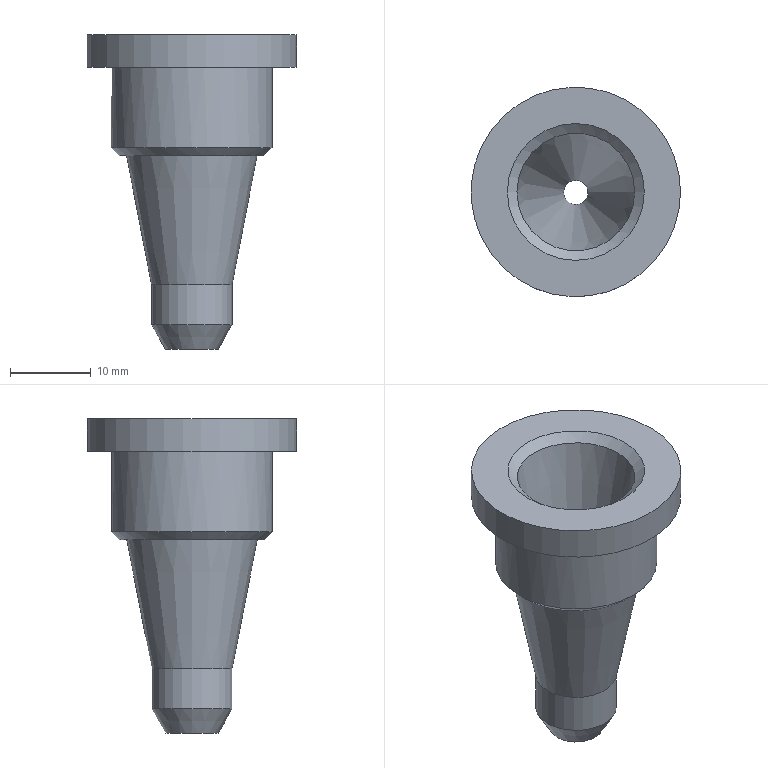Component | NX | SMALL_NOZZLE | 1 solid | 13 faces | box 26 x 26 x 39 mm | volume 5956 mm3 | cone 5 | plane 4 | cylinder 4 | commonest cylinder face diameters 10 x1 3 x1 26 x1 20 x1
STEP:
#1=CARTESIAN_POINT('',(0.,0.,0.));
#2=DIRECTION('',(0.,0.,1.));
#3=DIRECTION('',(1.,0.,0.));
#4=AXIS2_PLACEMENT_3D('',#1,#2,#3);
#5=CARTESIAN_POINT('',(1.284,5.784,7.));
#6=VERTEX_POINT('',#5);
#7=CARTESIAN_POINT('',(10.284,5.784,7.));
#8=DIRECTION('',(0.,0.,-1.));
#9=DIRECTION('',(-1.,0.,0.));
#10=AXIS2_PLACEMENT_3D('',#7,#8,#9);
#11=CIRCLE('',#10,9.);
#12=CARTESIAN_POINT('',(10.284,15.784,7.));
#13=DIRECTION('',(0.,0.,-1.));
#14=DIRECTION('',(-1.,0.,0.));
#15=AXIS2_PLACEMENT_3D('',#12,#13,#14);
#16=PLANE('',#15);
#17=CARTESIAN_POINT('',(0.,-10.));
#18=DIRECTION('',(1.,0.));
#19=AXIS2_PLACEMENT_2D('',#17,#18);
#20=CIRCLE('',#19,9.);
#21=(GEOMETRIC_REPRESENTATION_CONTEXT(2)PARAMETRIC_REPRESENTATION_CONTEXT()REPRESENTATION_CONTEXT('',''));
#22=DEFINITIONAL_REPRESENTATION('',(#20),#21);
#23=PCURVE('',#16,#22);
#24=CARTESIAN_POINT('',(10.284,5.784,8.));
#25=DIRECTION('',(0.,0.,1.));
#26=DIRECTION('',(1.,0.,0.));
#27=AXIS2_PLACEMENT_3D('',#24,#25,#26);
#28=CONICAL_SURFACE('',#27,10.,0.7854);
#29=CARTESIAN_POINT('',(9.425,-1.));
#30=DIRECTION('',(-1.,0.));
#31=VECTOR('',#30,1.);
#32=LINE('',#29,#31);
#33=(GEOMETRIC_REPRESENTATION_CONTEXT(2)PARAMETRIC_REPRESENTATION_CONTEXT()REPRESENTATION_CONTEXT('',''));
#34=DEFINITIONAL_REPRESENTATION('',(#32),#33);
#35=PCURVE('',#28,#34);
#36=SURFACE_CURVE('',#11,(#23,#35),.PCURVE_S1.);
#37=EDGE_CURVE('',#6,#6,#36,.T.);
#38=ORIENTED_EDGE('',*,*,#37,.T.);
#39=EDGE_LOOP('',(#38));
#40=FACE_BOUND('',#39,.T.);
#41=CARTESIAN_POINT('',(18.381,5.784,7.));
#42=VERTEX_POINT('',#41);
#43=CARTESIAN_POINT('',(10.284,5.784,7.));
#44=DIRECTION('',(0.,0.,1.));
#45=DIRECTION('',(1.,0.,0.));
#46=AXIS2_PLACEMENT_3D('',#43,#44,#45);
#47=CIRCLE('',#46,8.097);
#48=CARTESIAN_POINT('',(-8.097,-10.));
#49=CARTESIAN_POINT('',(-8.097,4.024));
#50=CARTESIAN_POINT('',(4.048,-2.988));
#51=CARTESIAN_POINT('',(16.194,-10.));
#52=CARTESIAN_POINT('',(4.048,-17.012));
#53=CARTESIAN_POINT('',(-8.097,-24.024));
#54=CARTESIAN_POINT('',(-8.097,-10.));
#55=(BOUNDED_CURVE()B_SPLINE_CURVE(2,(#48,#49,#50,#51,#52,#53,#54),.UNSPECIFIED.,.T.,.F.)B_SPLINE_CURVE_WITH_KNOTS((1,2,2,2,2,1),(-2.094,0.,2.094,4.189,6.283,8.378),.UNSPECIFIED.)CURVE()GEOMETRIC_REPRESENTATION_ITEM()RATIONAL_B_SPLINE_CURVE((1.,0.5,1.,0.5,1.,0.5,1.))REPRESENTATION_ITEM(''));
#56=(GEOMETRIC_REPRESENTATION_CONTEXT(2)PARAMETRIC_REPRESENTATION_CONTEXT()REPRESENTATION_CONTEXT('',''));
#57=DEFINITIONAL_REPRESENTATION('',(#55),#56);
#58=PCURVE('',#16,#57);
#59=CARTESIAN_POINT('',(10.284,5.784,7.));
#60=DIRECTION('',(0.,0.,1.));
#61=DIRECTION('',(1.,0.,0.));
#62=AXIS2_PLACEMENT_3D('',#59,#60,#61);
#63=CONICAL_SURFACE('',#62,8.097,0.1912);
#64=CARTESIAN_POINT('',(0.,0.));
#65=DIRECTION('',(1.,0.));
#66=VECTOR('',#65,1.);
#67=LINE('',#64,#66);
#68=(GEOMETRIC_REPRESENTATION_CONTEXT(2)PARAMETRIC_REPRESENTATION_CONTEXT()REPRESENTATION_CONTEXT('',''));
#69=DEFINITIONAL_REPRESENTATION('',(#67),#68);
#70=PCURVE('',#63,#69);
#71=SURFACE_CURVE('',#47,(#58,#70),.PCURVE_S1.);
#72=EDGE_CURVE('',#42,#42,#71,.T.);
#73=ORIENTED_EDGE('',*,*,#72,.T.);
#74=EDGE_LOOP('',(#73));
#75=FACE_BOUND('',#74,.T.);
#76=ADVANCED_FACE('',(#40,#75),#16,.T.);
#77=CARTESIAN_POINT('',(15.284,5.784,-9.));
#78=VERTEX_POINT('',#77);
#79=CARTESIAN_POINT('',(10.284,5.784,-9.));
#80=DIRECTION('',(0.,0.,1.));
#81=DIRECTION('',(1.,0.,0.));
#82=AXIS2_PLACEMENT_3D('',#79,#80,#81);
#83=CIRCLE('',#82,5.);
#84=CARTESIAN_POINT('',(0.,-16.));
#85=DIRECTION('',(1.,0.));
#86=VECTOR('',#85,1.);
#87=LINE('',#84,#86);
#88=(GEOMETRIC_REPRESENTATION_CONTEXT(2)PARAMETRIC_REPRESENTATION_CONTEXT()REPRESENTATION_CONTEXT('',''));
#89=DEFINITIONAL_REPRESENTATION('',(#87),#88);
#90=PCURVE('',#63,#89);
#91=CARTESIAN_POINT('',(10.284,5.784,22.));
#92=DIRECTION('',(0.,0.,1.));
#93=DIRECTION('',(1.,0.,0.));
#94=AXIS2_PLACEMENT_3D('',#91,#92,#93);
#95=CYLINDRICAL_SURFACE('',#94,5.);
#96=CARTESIAN_POINT('',(0.,-31.));
#97=DIRECTION('',(1.,0.));
#98=VECTOR('',#97,1.);
#99=LINE('',#96,#98);
#100=(GEOMETRIC_REPRESENTATION_CONTEXT(2)PARAMETRIC_REPRESENTATION_CONTEXT()REPRESENTATION_CONTEXT('',''));
#101=DEFINITIONAL_REPRESENTATION('',(#99),#100);
#102=PCURVE('',#95,#101);
#103=SURFACE_CURVE('',#83,(#90,#102),.PCURVE_S1.);
#104=EDGE_CURVE('',#78,#78,#103,.T.);
#105=ORIENTED_EDGE('',*,*,#104,.T.);
#106=CARTESIAN_POINT('',(15.284,5.784,-9.));
#107=CARTESIAN_POINT('',(18.381,5.784,7.));
#108=B_SPLINE_CURVE_WITH_KNOTS('',1,(#106,#107),.UNSPECIFIED.,.F.,.F.,(2,2),(-16.297,0.),.PIECEWISE_BEZIER_KNOTS.);
#109=CARTESIAN_POINT('',(6.283,0.));
#110=DIRECTION('',(0.,1.));
#111=VECTOR('',#110,1.);
#112=LINE('',#109,#111);
#113=(GEOMETRIC_REPRESENTATION_CONTEXT(2)PARAMETRIC_REPRESENTATION_CONTEXT()REPRESENTATION_CONTEXT('',''));
#114=DEFINITIONAL_REPRESENTATION('',(#112),#113);
#115=PCURVE('',#63,#114);
#116=CARTESIAN_POINT('',(0.,0.));
#117=DIRECTION('',(0.,1.));
#118=VECTOR('',#117,1.);
#119=LINE('',#116,#118);
#120=(GEOMETRIC_REPRESENTATION_CONTEXT(2)PARAMETRIC_REPRESENTATION_CONTEXT()REPRESENTATION_CONTEXT('',''));
#121=DEFINITIONAL_REPRESENTATION('',(#119),#120);
#122=PCURVE('',#63,#121);
#123=SEAM_CURVE('',#108,(#115,#122),.PCURVE_S1.);
#124=EDGE_CURVE('',#78,#42,#123,.T.);
#125=ORIENTED_EDGE('',*,*,#124,.T.);
#126=ORIENTED_EDGE('',*,*,#72,.F.);
#127=ORIENTED_EDGE('',*,*,#124,.F.);
#128=EDGE_LOOP('',(#105,#125,#126,#127));
#129=FACE_BOUND('',#128,.T.);
#130=ADVANCED_FACE('',(#129),#63,.T.);
#131=CARTESIAN_POINT('',(15.284,5.784,-14.));
#132=VERTEX_POINT('',#131);
#133=CARTESIAN_POINT('',(10.284,5.784,-14.));
#134=DIRECTION('',(0.,0.,1.));
#135=DIRECTION('',(1.,0.,0.));
#136=AXIS2_PLACEMENT_3D('',#133,#134,#135);
#137=CIRCLE('',#136,5.);
#138=CARTESIAN_POINT('',(0.,-36.));
#139=DIRECTION('',(1.,0.));
#140=VECTOR('',#139,1.);
#141=LINE('',#138,#140);
#142=(GEOMETRIC_REPRESENTATION_CONTEXT(2)PARAMETRIC_REPRESENTATION_CONTEXT()REPRESENTATION_CONTEXT('',''));
#143=DEFINITIONAL_REPRESENTATION('',(#141),#142);
#144=PCURVE('',#95,#143);
#145=CARTESIAN_POINT('',(10.284,5.784,-14.));
#146=DIRECTION('',(0.,0.,1.));
#147=DIRECTION('',(1.,0.,0.));
#148=AXIS2_PLACEMENT_3D('',#145,#146,#147);
#149=CONICAL_SURFACE('',#148,5.,0.5236);
#150=CARTESIAN_POINT('',(0.,-0.));
#151=DIRECTION('',(1.,0.));
#152=VECTOR('',#151,1.);
#153=LINE('',#150,#152);
#154=(GEOMETRIC_REPRESENTATION_CONTEXT(2)PARAMETRIC_REPRESENTATION_CONTEXT()REPRESENTATION_CONTEXT('',''));
#155=DEFINITIONAL_REPRESENTATION('',(#153),#154);
#156=PCURVE('',#149,#155);
#157=SURFACE_CURVE('',#137,(#144,#156),.PCURVE_S1.);
#158=EDGE_CURVE('',#132,#132,#157,.T.);
#159=ORIENTED_EDGE('',*,*,#158,.T.);
#160=CARTESIAN_POINT('',(15.284,5.784,-14.));
#161=CARTESIAN_POINT('',(15.284,5.784,-9.));
#162=B_SPLINE_CURVE_WITH_KNOTS('',1,(#160,#161),.UNSPECIFIED.,.F.,.F.,(2,2),(-36.,-31.),.PIECEWISE_BEZIER_KNOTS.);
#163=CARTESIAN_POINT('',(6.283,0.));
#164=DIRECTION('',(0.,1.));
#165=VECTOR('',#164,1.);
#166=LINE('',#163,#165);
#167=(GEOMETRIC_REPRESENTATION_CONTEXT(2)PARAMETRIC_REPRESENTATION_CONTEXT()REPRESENTATION_CONTEXT('',''));
#168=DEFINITIONAL_REPRESENTATION('',(#166),#167);
#169=PCURVE('',#95,#168);
#170=CARTESIAN_POINT('',(0.,0.));
#171=DIRECTION('',(0.,1.));
#172=VECTOR('',#171,1.);
#173=LINE('',#170,#172);
#174=(GEOMETRIC_REPRESENTATION_CONTEXT(2)PARAMETRIC_REPRESENTATION_CONTEXT()REPRESENTATION_CONTEXT('',''));
#175=DEFINITIONAL_REPRESENTATION('',(#173),#174);
#176=PCURVE('',#95,#175);
#177=SEAM_CURVE('',#162,(#169,#176),.PCURVE_S1.);
#178=EDGE_CURVE('',#132,#78,#177,.T.);
#179=ORIENTED_EDGE('',*,*,#178,.T.);
#180=ORIENTED_EDGE('',*,*,#104,.F.);
#181=ORIENTED_EDGE('',*,*,#178,.F.);
#182=EDGE_LOOP('',(#159,#179,#180,#181));
#183=FACE_BOUND('',#182,.T.);
#184=ADVANCED_FACE('',(#183),#95,.T.);
#185=CARTESIAN_POINT('',(13.552,5.784,-17.));
#186=VERTEX_POINT('',#185);
#187=CARTESIAN_POINT('',(10.284,5.784,-17.));
#188=DIRECTION('',(0.,0.,1.));
#189=DIRECTION('',(1.,0.,0.));
#190=AXIS2_PLACEMENT_3D('',#187,#188,#189);
#191=CIRCLE('',#190,3.268);
#192=CARTESIAN_POINT('',(0.,-3.));
#193=DIRECTION('',(1.,0.));
#194=VECTOR('',#193,1.);
#195=LINE('',#192,#194);
#196=(GEOMETRIC_REPRESENTATION_CONTEXT(2)PARAMETRIC_REPRESENTATION_CONTEXT()REPRESENTATION_CONTEXT('',''));
#197=DEFINITIONAL_REPRESENTATION('',(#195),#196);
#198=PCURVE('',#149,#197);
#199=CARTESIAN_POINT('',(10.284,9.052,-17.));
#200=DIRECTION('',(0.,0.,-1.));
#201=DIRECTION('',(-1.,0.,0.));
#202=AXIS2_PLACEMENT_3D('',#199,#200,#201);
#203=PLANE('',#202);
#204=CARTESIAN_POINT('',(-3.268,-3.268));
#205=CARTESIAN_POINT('',(-3.268,2.392));
#206=CARTESIAN_POINT('',(1.634,-0.4378));
#207=CARTESIAN_POINT('',(6.536,-3.268));
#208=CARTESIAN_POINT('',(1.634,-6.098));
#209=CARTESIAN_POINT('',(-3.268,-8.928));
#210=CARTESIAN_POINT('',(-3.268,-3.268));
#211=(BOUNDED_CURVE()B_SPLINE_CURVE(2,(#204,#205,#206,#207,#208,#209,#210),.UNSPECIFIED.,.T.,.F.)B_SPLINE_CURVE_WITH_KNOTS((1,2,2,2,2,1),(-2.094,0.,2.094,4.189,6.283,8.378),.UNSPECIFIED.)CURVE()GEOMETRIC_REPRESENTATION_ITEM()RATIONAL_B_SPLINE_CURVE((1.,0.5,1.,0.5,1.,0.5,1.))REPRESENTATION_ITEM(''));
#212=(GEOMETRIC_REPRESENTATION_CONTEXT(2)PARAMETRIC_REPRESENTATION_CONTEXT()REPRESENTATION_CONTEXT('',''));
#213=DEFINITIONAL_REPRESENTATION('',(#211),#212);
#214=PCURVE('',#203,#213);
#215=SURFACE_CURVE('',#191,(#198,#214),.PCURVE_S1.);
#216=EDGE_CURVE('',#186,#186,#215,.T.);
#217=ORIENTED_EDGE('',*,*,#216,.T.);
#218=CARTESIAN_POINT('',(13.552,5.784,-17.));
#219=CARTESIAN_POINT('',(15.284,5.784,-14.));
#220=B_SPLINE_CURVE_WITH_KNOTS('',1,(#218,#219),.UNSPECIFIED.,.F.,.F.,(2,2),(-3.464,-0.),.PIECEWISE_BEZIER_KNOTS.);
#221=CARTESIAN_POINT('',(6.283,0.));
#222=DIRECTION('',(0.,1.));
#223=VECTOR('',#222,1.);
#224=LINE('',#221,#223);
#225=(GEOMETRIC_REPRESENTATION_CONTEXT(2)PARAMETRIC_REPRESENTATION_CONTEXT()REPRESENTATION_CONTEXT('',''));
#226=DEFINITIONAL_REPRESENTATION('',(#224),#225);
#227=PCURVE('',#149,#226);
#228=CARTESIAN_POINT('',(0.,0.));
#229=DIRECTION('',(0.,1.));
#230=VECTOR('',#229,1.);
#231=LINE('',#228,#230);
#232=(GEOMETRIC_REPRESENTATION_CONTEXT(2)PARAMETRIC_REPRESENTATION_CONTEXT()REPRESENTATION_CONTEXT('',''));
#233=DEFINITIONAL_REPRESENTATION('',(#231),#232);
#234=PCURVE('',#149,#233);
#235=SEAM_CURVE('',#220,(#227,#234),.PCURVE_S1.);
#236=EDGE_CURVE('',#186,#132,#235,.T.);
#237=ORIENTED_EDGE('',*,*,#236,.T.);
#238=ORIENTED_EDGE('',*,*,#158,.F.);
#239=ORIENTED_EDGE('',*,*,#236,.F.);
#240=EDGE_LOOP('',(#217,#237,#238,#239));
#241=FACE_BOUND('',#240,.T.);
#242=ADVANCED_FACE('',(#241),#149,.T.);
#243=CARTESIAN_POINT('',(11.784,5.784,-17.));
#244=VERTEX_POINT('',#243);
#245=CARTESIAN_POINT('',(10.284,5.784,-17.));
#246=DIRECTION('',(0.,0.,1.));
#247=DIRECTION('',(1.,0.,0.));
#248=AXIS2_PLACEMENT_3D('',#245,#246,#247);
#249=CIRCLE('',#248,1.5);
#250=CARTESIAN_POINT('',(-1.5,-3.268));
#251=CARTESIAN_POINT('',(-1.5,-0.6699));
#252=CARTESIAN_POINT('',(0.75,-1.969));
#253=CARTESIAN_POINT('',(3.,-3.268));
#254=CARTESIAN_POINT('',(0.75,-4.567));
#255=CARTESIAN_POINT('',(-1.5,-5.866));
#256=CARTESIAN_POINT('',(-1.5,-3.268));
#257=(BOUNDED_CURVE()B_SPLINE_CURVE(2,(#250,#251,#252,#253,#254,#255,#256),.UNSPECIFIED.,.T.,.F.)B_SPLINE_CURVE_WITH_KNOTS((1,2,2,2,2,1),(-2.094,0.,2.094,4.189,6.283,8.378),.UNSPECIFIED.)CURVE()GEOMETRIC_REPRESENTATION_ITEM()RATIONAL_B_SPLINE_CURVE((1.,0.5,1.,0.5,1.,0.5,1.))REPRESENTATION_ITEM(''));
#258=(GEOMETRIC_REPRESENTATION_CONTEXT(2)PARAMETRIC_REPRESENTATION_CONTEXT()REPRESENTATION_CONTEXT('',''));
#259=DEFINITIONAL_REPRESENTATION('',(#257),#258);
#260=PCURVE('',#203,#259);
#261=CARTESIAN_POINT('',(10.284,5.784,22.));
#262=DIRECTION('',(0.,0.,1.));
#263=DIRECTION('',(1.,0.,0.));
#264=AXIS2_PLACEMENT_3D('',#261,#262,#263);
#265=CYLINDRICAL_SURFACE('',#264,1.5);
#266=CARTESIAN_POINT('',(0.,-39.));
#267=DIRECTION('',(1.,0.));
#268=VECTOR('',#267,1.);
#269=LINE('',#266,#268);
#270=(GEOMETRIC_REPRESENTATION_CONTEXT(2)PARAMETRIC_REPRESENTATION_CONTEXT()REPRESENTATION_CONTEXT('',''));
#271=DEFINITIONAL_REPRESENTATION('',(#269),#270);
#272=PCURVE('',#265,#271);
#273=SURFACE_CURVE('',#249,(#260,#272),.PCURVE_S1.);
#274=EDGE_CURVE('',#244,#244,#273,.T.);
#275=ORIENTED_EDGE('',*,*,#274,.T.);
#276=EDGE_LOOP('',(#275));
#277=FACE_BOUND('',#276,.T.);
#278=ORIENTED_EDGE('',*,*,#216,.F.);
#279=EDGE_LOOP('',(#278));
#280=FACE_BOUND('',#279,.T.);
#281=ADVANCED_FACE('',(#277,#280),#203,.T.);
#282=CARTESIAN_POINT('',(11.784,5.784,-9.));
#283=VERTEX_POINT('',#282);
#284=CARTESIAN_POINT('',(10.284,5.784,-9.));
#285=DIRECTION('',(0.,0.,1.));
#286=DIRECTION('',(1.,0.,0.));
#287=AXIS2_PLACEMENT_3D('',#284,#285,#286);
#288=CIRCLE('',#287,1.5);
#289=CARTESIAN_POINT('',(0.,-31.));
#290=DIRECTION('',(1.,0.));
#291=VECTOR('',#290,1.);
#292=LINE('',#289,#291);
#293=(GEOMETRIC_REPRESENTATION_CONTEXT(2)PARAMETRIC_REPRESENTATION_CONTEXT()REPRESENTATION_CONTEXT('',''));
#294=DEFINITIONAL_REPRESENTATION('',(#292),#293);
#295=PCURVE('',#265,#294);
#296=CARTESIAN_POINT('',(10.284,5.784,-9.));
#297=DIRECTION('',(0.,0.,1.));
#298=DIRECTION('',(1.,0.,0.));
#299=AXIS2_PLACEMENT_3D('',#296,#297,#298);
#300=CONICAL_SURFACE('',#299,1.5,0.1912);
#301=CARTESIAN_POINT('',(0.,0.));
#302=DIRECTION('',(1.,0.));
#303=VECTOR('',#302,1.);
#304=LINE('',#301,#303);
#305=(GEOMETRIC_REPRESENTATION_CONTEXT(2)PARAMETRIC_REPRESENTATION_CONTEXT()REPRESENTATION_CONTEXT('',''));
#306=DEFINITIONAL_REPRESENTATION('',(#304),#305);
#307=PCURVE('',#300,#306);
#308=SURFACE_CURVE('',#288,(#295,#307),.PCURVE_S1.);
#309=EDGE_CURVE('',#283,#283,#308,.T.);
#310=ORIENTED_EDGE('',*,*,#309,.F.);
#311=CARTESIAN_POINT('',(11.784,5.784,-17.));
#312=CARTESIAN_POINT('',(11.784,5.784,-9.));
#313=B_SPLINE_CURVE_WITH_KNOTS('',1,(#311,#312),.UNSPECIFIED.,.F.,.F.,(2,2),(-39.,-31.),.PIECEWISE_BEZIER_KNOTS.);
#314=CARTESIAN_POINT('',(0.,0.));
#315=DIRECTION('',(0.,1.));
#316=VECTOR('',#315,1.);
#317=LINE('',#314,#316);
#318=(GEOMETRIC_REPRESENTATION_CONTEXT(2)PARAMETRIC_REPRESENTATION_CONTEXT()REPRESENTATION_CONTEXT('',''));
#319=DEFINITIONAL_REPRESENTATION('',(#317),#318);
#320=PCURVE('',#265,#319);
#321=CARTESIAN_POINT('',(6.283,0.));
#322=DIRECTION('',(0.,1.));
#323=VECTOR('',#322,1.);
#324=LINE('',#321,#323);
#325=(GEOMETRIC_REPRESENTATION_CONTEXT(2)PARAMETRIC_REPRESENTATION_CONTEXT()REPRESENTATION_CONTEXT('',''));
#326=DEFINITIONAL_REPRESENTATION('',(#324),#325);
#327=PCURVE('',#265,#326);
#328=SEAM_CURVE('',#313,(#320,#327),.PCURVE_S1.);
#329=EDGE_CURVE('',#244,#283,#328,.T.);
#330=ORIENTED_EDGE('',*,*,#329,.F.);
#331=ORIENTED_EDGE('',*,*,#274,.T.);
#332=ORIENTED_EDGE('',*,*,#329,.T.);
#333=EDGE_LOOP('',(#310,#330,#331,#332));
#334=FACE_BOUND('',#333,.F.);
#335=ADVANCED_FACE('',(#334),#265,.F.);
#336=CARTESIAN_POINT('',(17.594,5.784,21.018));
#337=VERTEX_POINT('',#336);
#338=CARTESIAN_POINT('',(2.974,5.784,21.018));
#339=VERTEX_POINT('',#338);
#340=CARTESIAN_POINT('',(10.284,5.784,21.018));
#341=DIRECTION('',(0.,0.,1.));
#342=DIRECTION('',(-1.,0.,0.));
#343=AXIS2_PLACEMENT_3D('',#340,#341,#342);
#344=CIRCLE('',#343,7.31);
#345=CARTESIAN_POINT('',(-3.142,30.018));
#346=DIRECTION('',(1.,0.));
#347=VECTOR('',#346,1.);
#348=LINE('',#345,#347);
#349=(GEOMETRIC_REPRESENTATION_CONTEXT(2)PARAMETRIC_REPRESENTATION_CONTEXT()REPRESENTATION_CONTEXT('',''));
#350=DEFINITIONAL_REPRESENTATION('',(#348),#349);
#351=PCURVE('',#300,#350);
#352=CARTESIAN_POINT('',(10.284,5.784,21.018));
#353=DIRECTION('',(0.,0.,1.));
#354=DIRECTION('',(1.,0.,0.));
#355=AXIS2_PLACEMENT_3D('',#352,#353,#354);
#356=CONICAL_SURFACE('',#355,7.31,0.881);
#357=CARTESIAN_POINT('',(-3.142,0.));
#358=DIRECTION('',(1.,-0.));
#359=VECTOR('',#358,1.);
#360=LINE('',#357,#359);
#361=(GEOMETRIC_REPRESENTATION_CONTEXT(2)PARAMETRIC_REPRESENTATION_CONTEXT()REPRESENTATION_CONTEXT('',''));
#362=DEFINITIONAL_REPRESENTATION('',(#360),#361);
#363=PCURVE('',#356,#362);
#364=SURFACE_CURVE('',#344,(#351,#363),.PCURVE_S1.);
#365=EDGE_CURVE('',#337,#339,#364,.T.);
#366=ORIENTED_EDGE('',*,*,#365,.F.);
#367=CARTESIAN_POINT('',(11.784,5.784,-9.));
#368=CARTESIAN_POINT('',(17.594,5.784,21.018));
#369=B_SPLINE_CURVE_WITH_KNOTS('',1,(#367,#368),.UNSPECIFIED.,.F.,.F.,(2,2),(0.,30.575),.PIECEWISE_BEZIER_KNOTS.);
#370=CARTESIAN_POINT('',(0.,0.));
#371=DIRECTION('',(0.,1.));
#372=VECTOR('',#371,1.);
#373=LINE('',#370,#372);
#374=(GEOMETRIC_REPRESENTATION_CONTEXT(2)PARAMETRIC_REPRESENTATION_CONTEXT()REPRESENTATION_CONTEXT('',''));
#375=DEFINITIONAL_REPRESENTATION('',(#373),#374);
#376=PCURVE('',#300,#375);
#377=CARTESIAN_POINT('',(6.283,0.));
#378=DIRECTION('',(0.,1.));
#379=VECTOR('',#378,1.);
#380=LINE('',#377,#379);
#381=(GEOMETRIC_REPRESENTATION_CONTEXT(2)PARAMETRIC_REPRESENTATION_CONTEXT()REPRESENTATION_CONTEXT('',''));
#382=DEFINITIONAL_REPRESENTATION('',(#380),#381);
#383=PCURVE('',#300,#382);
#384=SEAM_CURVE('',#369,(#376,#383),.PCURVE_S1.);
#385=EDGE_CURVE('',#283,#337,#384,.T.);
#386=ORIENTED_EDGE('',*,*,#385,.F.);
#387=ORIENTED_EDGE('',*,*,#309,.T.);
#388=ORIENTED_EDGE('',*,*,#385,.T.);
#389=CARTESIAN_POINT('',(10.284,5.784,21.018));
#390=DIRECTION('',(0.,0.,1.));
#391=DIRECTION('',(-1.,0.,0.));
#392=AXIS2_PLACEMENT_3D('',#389,#390,#391);
#393=CIRCLE('',#392,7.31);
#394=CARTESIAN_POINT('',(3.142,30.018));
#395=DIRECTION('',(1.,0.));
#396=VECTOR('',#395,1.);
#397=LINE('',#394,#396);
#398=(GEOMETRIC_REPRESENTATION_CONTEXT(2)PARAMETRIC_REPRESENTATION_CONTEXT()REPRESENTATION_CONTEXT('',''));
#399=DEFINITIONAL_REPRESENTATION('',(#397),#398);
#400=PCURVE('',#300,#399);
#401=CARTESIAN_POINT('',(3.142,0.));
#402=DIRECTION('',(1.,0.));
#403=VECTOR('',#402,1.);
#404=LINE('',#401,#403);
#405=(GEOMETRIC_REPRESENTATION_CONTEXT(2)PARAMETRIC_REPRESENTATION_CONTEXT()REPRESENTATION_CONTEXT('',''));
#406=DEFINITIONAL_REPRESENTATION('',(#404),#405);
#407=PCURVE('',#356,#406);
#408=SURFACE_CURVE('',#393,(#400,#407),.PCURVE_S1.);
#409=EDGE_CURVE('',#339,#337,#408,.T.);
#410=ORIENTED_EDGE('',*,*,#409,.F.);
#411=EDGE_LOOP('',(#366,#386,#387,#388,#410));
#412=FACE_BOUND('',#411,.F.);
#413=ADVANCED_FACE('',(#412),#300,.F.);
#414=CARTESIAN_POINT('',(18.784,5.784,22.));
#415=VERTEX_POINT('',#414);
#416=CARTESIAN_POINT('',(10.284,5.784,22.));
#417=DIRECTION('',(0.,0.,-1.));
#418=DIRECTION('',(1.,0.,0.));
#419=AXIS2_PLACEMENT_3D('',#416,#417,#418);
#420=CIRCLE('',#419,8.5);
#421=CARTESIAN_POINT('',(10.284,13.284,22.));
#422=DIRECTION('',(0.,0.,1.));
#423=DIRECTION('',(1.,0.,0.));
#424=AXIS2_PLACEMENT_3D('',#421,#422,#423);
#425=PLANE('',#424);
#426=CARTESIAN_POINT('',(8.5,-7.5));
#427=CARTESIAN_POINT('',(8.5,-22.222));
#428=CARTESIAN_POINT('',(-4.25,-14.861));
#429=CARTESIAN_POINT('',(-17.,-7.5));
#430=CARTESIAN_POINT('',(-4.25,-0.1388));
#431=CARTESIAN_POINT('',(8.5,7.222));
#432=CARTESIAN_POINT('',(8.5,-7.5));
#433=(BOUNDED_CURVE()B_SPLINE_CURVE(2,(#426,#427,#428,#429,#430,#431,#432),.UNSPECIFIED.,.T.,.F.)B_SPLINE_CURVE_WITH_KNOTS((1,2,2,2,2,1),(-2.094,0.,2.094,4.189,6.283,8.378),.UNSPECIFIED.)CURVE()GEOMETRIC_REPRESENTATION_ITEM()RATIONAL_B_SPLINE_CURVE((1.,0.5,1.,0.5,1.,0.5,1.))REPRESENTATION_ITEM(''));
#434=(GEOMETRIC_REPRESENTATION_CONTEXT(2)PARAMETRIC_REPRESENTATION_CONTEXT()REPRESENTATION_CONTEXT('',''));
#435=DEFINITIONAL_REPRESENTATION('',(#433),#434);
#436=PCURVE('',#425,#435);
#437=CARTESIAN_POINT('',(6.283,0.9818));
#438=DIRECTION('',(-1.,0.));
#439=VECTOR('',#438,1.);
#440=LINE('',#437,#439);
#441=(GEOMETRIC_REPRESENTATION_CONTEXT(2)PARAMETRIC_REPRESENTATION_CONTEXT()REPRESENTATION_CONTEXT('',''));
#442=DEFINITIONAL_REPRESENTATION('',(#440),#441);
#443=PCURVE('',#356,#442);
#444=SURFACE_CURVE('',#420,(#436,#443),.PCURVE_S1.);
#445=EDGE_CURVE('',#415,#415,#444,.T.);
#446=ORIENTED_EDGE('',*,*,#445,.T.);
#447=EDGE_LOOP('',(#446));
#448=FACE_BOUND('',#447,.T.);
#449=CARTESIAN_POINT('',(23.284,5.784,22.));
#450=VERTEX_POINT('',#449);
#451=CARTESIAN_POINT('',(10.284,5.784,22.));
#452=DIRECTION('',(0.,0.,1.));
#453=DIRECTION('',(1.,0.,0.));
#454=AXIS2_PLACEMENT_3D('',#451,#452,#453);
#455=CIRCLE('',#454,13.);
#456=CARTESIAN_POINT('',(0.,-7.5));
#457=DIRECTION('',(1.,0.));
#458=AXIS2_PLACEMENT_2D('',#456,#457);
#459=CIRCLE('',#458,13.);
#460=(GEOMETRIC_REPRESENTATION_CONTEXT(2)PARAMETRIC_REPRESENTATION_CONTEXT()REPRESENTATION_CONTEXT('',''));
#461=DEFINITIONAL_REPRESENTATION('',(#459),#460);
#462=PCURVE('',#425,#461);
#463=CARTESIAN_POINT('',(10.284,5.784,22.));
#464=DIRECTION('',(0.,0.,1.));
#465=DIRECTION('',(1.,0.,0.));
#466=AXIS2_PLACEMENT_3D('',#463,#464,#465);
#467=CYLINDRICAL_SURFACE('',#466,13.);
#468=CARTESIAN_POINT('',(0.,0.));
#469=DIRECTION('',(1.,0.));
#470=VECTOR('',#469,1.);
#471=LINE('',#468,#470);
#472=(GEOMETRIC_REPRESENTATION_CONTEXT(2)PARAMETRIC_REPRESENTATION_CONTEXT()REPRESENTATION_CONTEXT('',''));
#473=DEFINITIONAL_REPRESENTATION('',(#471),#472);
#474=PCURVE('',#467,#473);
#475=SURFACE_CURVE('',#455,(#462,#474),.PCURVE_S1.);
#476=EDGE_CURVE('',#450,#450,#475,.T.);
#477=ORIENTED_EDGE('',*,*,#476,.T.);
#478=EDGE_LOOP('',(#477));
#479=FACE_BOUND('',#478,.T.);
#480=ADVANCED_FACE('',(#448,#479),#425,.T.);
#481=CARTESIAN_POINT('',(23.284,5.784,18.));
#482=VERTEX_POINT('',#481);
#483=CARTESIAN_POINT('',(10.284,5.784,18.));
#484=DIRECTION('',(0.,0.,1.));
#485=DIRECTION('',(1.,0.,0.));
#486=AXIS2_PLACEMENT_3D('',#483,#484,#485);
#487=CIRCLE('',#486,13.);
#488=CARTESIAN_POINT('',(0.,-4.));
#489=DIRECTION('',(1.,0.));
#490=VECTOR('',#489,1.);
#491=LINE('',#488,#490);
#492=(GEOMETRIC_REPRESENTATION_CONTEXT(2)PARAMETRIC_REPRESENTATION_CONTEXT()REPRESENTATION_CONTEXT('',''));
#493=DEFINITIONAL_REPRESENTATION('',(#491),#492);
#494=PCURVE('',#467,#493);
#495=CARTESIAN_POINT('',(10.284,18.784,18.));
#496=DIRECTION('',(0.,0.,-1.));
#497=DIRECTION('',(-1.,0.,0.));
#498=AXIS2_PLACEMENT_3D('',#495,#496,#497);
#499=PLANE('',#498);
#500=CARTESIAN_POINT('',(-13.,-13.));
#501=CARTESIAN_POINT('',(-13.,9.517));
#502=CARTESIAN_POINT('',(6.5,-1.742));
#503=CARTESIAN_POINT('',(26.,-13.));
#504=CARTESIAN_POINT('',(6.5,-24.258));
#505=CARTESIAN_POINT('',(-13.,-35.517));
#506=CARTESIAN_POINT('',(-13.,-13.));
#507=(BOUNDED_CURVE()B_SPLINE_CURVE(2,(#500,#501,#502,#503,#504,#505,#506),.UNSPECIFIED.,.T.,.F.)B_SPLINE_CURVE_WITH_KNOTS((1,2,2,2,2,1),(-2.094,0.,2.094,4.189,6.283,8.378),.UNSPECIFIED.)CURVE()GEOMETRIC_REPRESENTATION_ITEM()RATIONAL_B_SPLINE_CURVE((1.,0.5,1.,0.5,1.,0.5,1.))REPRESENTATION_ITEM(''));
#508=(GEOMETRIC_REPRESENTATION_CONTEXT(2)PARAMETRIC_REPRESENTATION_CONTEXT()REPRESENTATION_CONTEXT('',''));
#509=DEFINITIONAL_REPRESENTATION('',(#507),#508);
#510=PCURVE('',#499,#509);
#511=SURFACE_CURVE('',#487,(#494,#510),.PCURVE_S1.);
#512=EDGE_CURVE('',#482,#482,#511,.T.);
#513=ORIENTED_EDGE('',*,*,#512,.T.);
#514=CARTESIAN_POINT('',(23.284,5.784,18.));
#515=CARTESIAN_POINT('',(23.284,5.784,22.));
#516=B_SPLINE_CURVE_WITH_KNOTS('',1,(#514,#515),.UNSPECIFIED.,.F.,.F.,(2,2),(-4.,0.),.PIECEWISE_BEZIER_KNOTS.);
#517=CARTESIAN_POINT('',(6.283,0.));
#518=DIRECTION('',(0.,1.));
#519=VECTOR('',#518,1.);
#520=LINE('',#517,#519);
#521=(GEOMETRIC_REPRESENTATION_CONTEXT(2)PARAMETRIC_REPRESENTATION_CONTEXT()REPRESENTATION_CONTEXT('',''));
#522=DEFINITIONAL_REPRESENTATION('',(#520),#521);
#523=PCURVE('',#467,#522);
#524=CARTESIAN_POINT('',(0.,0.));
#525=DIRECTION('',(0.,1.));
#526=VECTOR('',#525,1.);
#527=LINE('',#524,#526);
#528=(GEOMETRIC_REPRESENTATION_CONTEXT(2)PARAMETRIC_REPRESENTATION_CONTEXT()REPRESENTATION_CONTEXT('',''));
#529=DEFINITIONAL_REPRESENTATION('',(#527),#528);
#530=PCURVE('',#467,#529);
#531=SEAM_CURVE('',#516,(#523,#530),.PCURVE_S1.);
#532=EDGE_CURVE('',#482,#450,#531,.T.);
#533=ORIENTED_EDGE('',*,*,#532,.T.);
#534=ORIENTED_EDGE('',*,*,#476,.F.);
#535=ORIENTED_EDGE('',*,*,#532,.F.);
#536=EDGE_LOOP('',(#513,#533,#534,#535));
#537=FACE_BOUND('',#536,.T.);
#538=ADVANCED_FACE('',(#537),#467,.T.);
#539=CARTESIAN_POINT('',(20.284,5.784,18.));
#540=VERTEX_POINT('',#539);
#541=CARTESIAN_POINT('',(10.284,5.784,18.));
#542=DIRECTION('',(0.,0.,1.));
#543=DIRECTION('',(1.,0.,0.));
#544=AXIS2_PLACEMENT_3D('',#541,#542,#543);
#545=CIRCLE('',#544,10.);
#546=CARTESIAN_POINT('',(-10.,-13.));
#547=CARTESIAN_POINT('',(-10.,4.321));
#548=CARTESIAN_POINT('',(5.,-4.34));
#549=CARTESIAN_POINT('',(20.,-13.));
#550=CARTESIAN_POINT('',(5.,-21.66));
#551=CARTESIAN_POINT('',(-10.,-30.321));
#552=CARTESIAN_POINT('',(-10.,-13.));
#553=(BOUNDED_CURVE()B_SPLINE_CURVE(2,(#546,#547,#548,#549,#550,#551,#552),.UNSPECIFIED.,.T.,.F.)B_SPLINE_CURVE_WITH_KNOTS((1,2,2,2,2,1),(-2.094,0.,2.094,4.189,6.283,8.378),.UNSPECIFIED.)CURVE()GEOMETRIC_REPRESENTATION_ITEM()RATIONAL_B_SPLINE_CURVE((1.,0.5,1.,0.5,1.,0.5,1.))REPRESENTATION_ITEM(''));
#554=(GEOMETRIC_REPRESENTATION_CONTEXT(2)PARAMETRIC_REPRESENTATION_CONTEXT()REPRESENTATION_CONTEXT('',''));
#555=DEFINITIONAL_REPRESENTATION('',(#553),#554);
#556=PCURVE('',#499,#555);
#557=CARTESIAN_POINT('',(10.284,5.784,22.));
#558=DIRECTION('',(0.,0.,1.));
#559=DIRECTION('',(1.,0.,0.));
#560=AXIS2_PLACEMENT_3D('',#557,#558,#559);
#561=CYLINDRICAL_SURFACE('',#560,10.);
#562=CARTESIAN_POINT('',(0.,-4.));
#563=DIRECTION('',(1.,0.));
#564=VECTOR('',#563,1.);
#565=LINE('',#562,#564);
#566=(GEOMETRIC_REPRESENTATION_CONTEXT(2)PARAMETRIC_REPRESENTATION_CONTEXT()REPRESENTATION_CONTEXT('',''));
#567=DEFINITIONAL_REPRESENTATION('',(#565),#566);
#568=PCURVE('',#561,#567);
#569=SURFACE_CURVE('',#545,(#556,#568),.PCURVE_S1.);
#570=EDGE_CURVE('',#540,#540,#569,.T.);
#571=ORIENTED_EDGE('',*,*,#570,.T.);
#572=EDGE_LOOP('',(#571));
#573=FACE_BOUND('',#572,.T.);
#574=ORIENTED_EDGE('',*,*,#512,.F.);
#575=EDGE_LOOP('',(#574));
#576=FACE_BOUND('',#575,.T.);
#577=ADVANCED_FACE('',(#573,#576),#499,.T.);
#578=CARTESIAN_POINT('',(0.2843,5.784,8.));
#579=VERTEX_POINT('',#578);
#580=CARTESIAN_POINT('',(20.284,5.784,8.));
#581=VERTEX_POINT('',#580);
#582=CARTESIAN_POINT('',(10.284,5.784,8.));
#583=DIRECTION('',(0.,0.,1.));
#584=DIRECTION('',(-1.,0.,0.));
#585=AXIS2_PLACEMENT_3D('',#582,#583,#584);
#586=CIRCLE('',#585,10.);
#587=CARTESIAN_POINT('',(3.142,-14.));
#588=DIRECTION('',(1.,0.));
#589=VECTOR('',#588,1.);
#590=LINE('',#587,#589);
#591=(GEOMETRIC_REPRESENTATION_CONTEXT(2)PARAMETRIC_REPRESENTATION_CONTEXT()REPRESENTATION_CONTEXT('',''));
#592=DEFINITIONAL_REPRESENTATION('',(#590),#591);
#593=PCURVE('',#561,#592);
#594=CARTESIAN_POINT('',(3.142,0.));
#595=DIRECTION('',(1.,0.));
#596=VECTOR('',#595,1.);
#597=LINE('',#594,#596);
#598=(GEOMETRIC_REPRESENTATION_CONTEXT(2)PARAMETRIC_REPRESENTATION_CONTEXT()REPRESENTATION_CONTEXT('',''));
#599=DEFINITIONAL_REPRESENTATION('',(#597),#598);
#600=PCURVE('',#28,#599);
#601=SURFACE_CURVE('',#586,(#593,#600),.PCURVE_S1.);
#602=EDGE_CURVE('',#579,#581,#601,.T.);
#603=ORIENTED_EDGE('',*,*,#602,.T.);
#604=CARTESIAN_POINT('',(20.284,5.784,8.));
#605=CARTESIAN_POINT('',(20.284,5.784,18.));
#606=B_SPLINE_CURVE_WITH_KNOTS('',1,(#604,#605),.UNSPECIFIED.,.F.,.F.,(2,2),(-14.,-4.),.PIECEWISE_BEZIER_KNOTS.);
#607=CARTESIAN_POINT('',(6.283,0.));
#608=DIRECTION('',(0.,1.));
#609=VECTOR('',#608,1.);
#610=LINE('',#607,#609);
#611=(GEOMETRIC_REPRESENTATION_CONTEXT(2)PARAMETRIC_REPRESENTATION_CONTEXT()REPRESENTATION_CONTEXT('',''));
#612=DEFINITIONAL_REPRESENTATION('',(#610),#611);
#613=PCURVE('',#561,#612);
#614=CARTESIAN_POINT('',(0.,0.));
#615=DIRECTION('',(0.,1.));
#616=VECTOR('',#615,1.);
#617=LINE('',#614,#616);
#618=(GEOMETRIC_REPRESENTATION_CONTEXT(2)PARAMETRIC_REPRESENTATION_CONTEXT()REPRESENTATION_CONTEXT('',''));
#619=DEFINITIONAL_REPRESENTATION('',(#617),#618);
#620=PCURVE('',#561,#619);
#621=SEAM_CURVE('',#606,(#613,#620),.PCURVE_S1.);
#622=EDGE_CURVE('',#581,#540,#621,.T.);
#623=ORIENTED_EDGE('',*,*,#622,.T.);
#624=ORIENTED_EDGE('',*,*,#570,.F.);
#625=ORIENTED_EDGE('',*,*,#622,.F.);
#626=CARTESIAN_POINT('',(10.284,5.784,8.));
#627=DIRECTION('',(0.,0.,1.));
#628=DIRECTION('',(-1.,0.,0.));
#629=AXIS2_PLACEMENT_3D('',#626,#627,#628);
#630=CIRCLE('',#629,10.);
#631=CARTESIAN_POINT('',(-3.142,-14.));
#632=DIRECTION('',(1.,0.));
#633=VECTOR('',#632,1.);
#634=LINE('',#631,#633);
#635=(GEOMETRIC_REPRESENTATION_CONTEXT(2)PARAMETRIC_REPRESENTATION_CONTEXT()REPRESENTATION_CONTEXT('',''));
#636=DEFINITIONAL_REPRESENTATION('',(#634),#635);
#637=PCURVE('',#561,#636);
#638=CARTESIAN_POINT('',(3.142,0.));
#639=DIRECTION('',(1.,-0.));
#640=VECTOR('',#639,1.);
#641=LINE('',#638,#640);
#642=(GEOMETRIC_REPRESENTATION_CONTEXT(2)PARAMETRIC_REPRESENTATION_CONTEXT()REPRESENTATION_CONTEXT('',''));
#643=DEFINITIONAL_REPRESENTATION('',(#641),#642);
#644=PCURVE('',#28,#643);
#645=SURFACE_CURVE('',#630,(#637,#644),.PCURVE_S1.);
#646=EDGE_CURVE('',#581,#579,#645,.T.);
#647=ORIENTED_EDGE('',*,*,#646,.T.);
#648=EDGE_LOOP('',(#603,#623,#624,#625,#647));
#649=FACE_BOUND('',#648,.T.);
#650=ADVANCED_FACE('',(#649),#561,.T.);
#651=ORIENTED_EDGE('',*,*,#445,.T.);
#652=CARTESIAN_POINT('',(17.594,5.784,21.018));
#653=CARTESIAN_POINT('',(18.784,5.784,22.));
#654=B_SPLINE_CURVE_WITH_KNOTS('',1,(#652,#653),.UNSPECIFIED.,.F.,.F.,(2,2),(0.,1.543),.PIECEWISE_BEZIER_KNOTS.);
#655=CARTESIAN_POINT('',(0.,0.));
#656=DIRECTION('',(0.,1.));
#657=VECTOR('',#656,1.);
#658=LINE('',#655,#657);
#659=(GEOMETRIC_REPRESENTATION_CONTEXT(2)PARAMETRIC_REPRESENTATION_CONTEXT()REPRESENTATION_CONTEXT('',''));
#660=DEFINITIONAL_REPRESENTATION('',(#658),#659);
#661=PCURVE('',#356,#660);
#662=CARTESIAN_POINT('',(6.283,0.));
#663=DIRECTION('',(0.,1.));
#664=VECTOR('',#663,1.);
#665=LINE('',#662,#664);
#666=(GEOMETRIC_REPRESENTATION_CONTEXT(2)PARAMETRIC_REPRESENTATION_CONTEXT()REPRESENTATION_CONTEXT('',''));
#667=DEFINITIONAL_REPRESENTATION('',(#665),#666);
#668=PCURVE('',#356,#667);
#669=SEAM_CURVE('',#654,(#661,#668),.PCURVE_S1.);
#670=EDGE_CURVE('',#337,#415,#669,.T.);
#671=ORIENTED_EDGE('',*,*,#670,.F.);
#672=ORIENTED_EDGE('',*,*,#365,.T.);
#673=ORIENTED_EDGE('',*,*,#409,.T.);
#674=ORIENTED_EDGE('',*,*,#670,.T.);
#675=EDGE_LOOP('',(#651,#671,#672,#673,#674));
#676=FACE_BOUND('',#675,.F.);
#677=ADVANCED_FACE('',(#676),#356,.F.);
#678=ORIENTED_EDGE('',*,*,#37,.F.);
#679=CARTESIAN_POINT('',(1.284,5.784,7.));
#680=CARTESIAN_POINT('',(0.2843,5.784,8.));
#681=B_SPLINE_CURVE_WITH_KNOTS('',1,(#679,#680),.UNSPECIFIED.,.F.,.F.,(2,2),(-1.414,0.),.PIECEWISE_BEZIER_KNOTS.);
#682=CARTESIAN_POINT('',(9.425,0.));
#683=DIRECTION('',(0.,1.));
#684=VECTOR('',#683,1.);
#685=LINE('',#682,#684);
#686=(GEOMETRIC_REPRESENTATION_CONTEXT(2)PARAMETRIC_REPRESENTATION_CONTEXT()REPRESENTATION_CONTEXT('',''));
#687=DEFINITIONAL_REPRESENTATION('',(#685),#686);
#688=PCURVE('',#28,#687);
#689=CARTESIAN_POINT('',(3.142,0.));
#690=DIRECTION('',(0.,1.));
#691=VECTOR('',#690,1.);
#692=LINE('',#689,#691);
#693=(GEOMETRIC_REPRESENTATION_CONTEXT(2)PARAMETRIC_REPRESENTATION_CONTEXT()REPRESENTATION_CONTEXT('',''));
#694=DEFINITIONAL_REPRESENTATION('',(#692),#693);
#695=PCURVE('',#28,#694);
#696=SEAM_CURVE('',#681,(#688,#695),.PCURVE_S1.);
#697=EDGE_CURVE('',#6,#579,#696,.T.);
#698=ORIENTED_EDGE('',*,*,#697,.T.);
#699=ORIENTED_EDGE('',*,*,#646,.F.);
#700=ORIENTED_EDGE('',*,*,#602,.F.);
#701=ORIENTED_EDGE('',*,*,#697,.F.);
#702=EDGE_LOOP('',(#678,#698,#699,#700,#701));
#703=FACE_BOUND('',#702,.T.);
#704=ADVANCED_FACE('',(#703),#28,.T.);
#705=CLOSED_SHELL('',(#76,#130,#184,#242,#281,#335,#413,#480,#538,#577,#650,#677,#704));
#706=MANIFOLD_SOLID_BREP('',#705);
#707=(LENGTH_UNIT()NAMED_UNIT(*)SI_UNIT(.MILLI.,.METRE.));
#708=UNCERTAINTY_MEASURE_WITH_UNIT(LENGTH_MEASURE(0.00001),#707,'','');
#709=(NAMED_UNIT(*)PLANE_ANGLE_UNIT()SI_UNIT($,.RADIAN.));
#710=(NAMED_UNIT(*)SI_UNIT($,.STERADIAN.)SOLID_ANGLE_UNIT());
#711=(GEOMETRIC_REPRESENTATION_CONTEXT(3)GLOBAL_UNCERTAINTY_ASSIGNED_CONTEXT((#708))GLOBAL_UNIT_ASSIGNED_CONTEXT((#707,#709,#710))REPRESENTATION_CONTEXT('',''));
#712=ADVANCED_BREP_SHAPE_REPRESENTATION('',(#4,#706),#711);